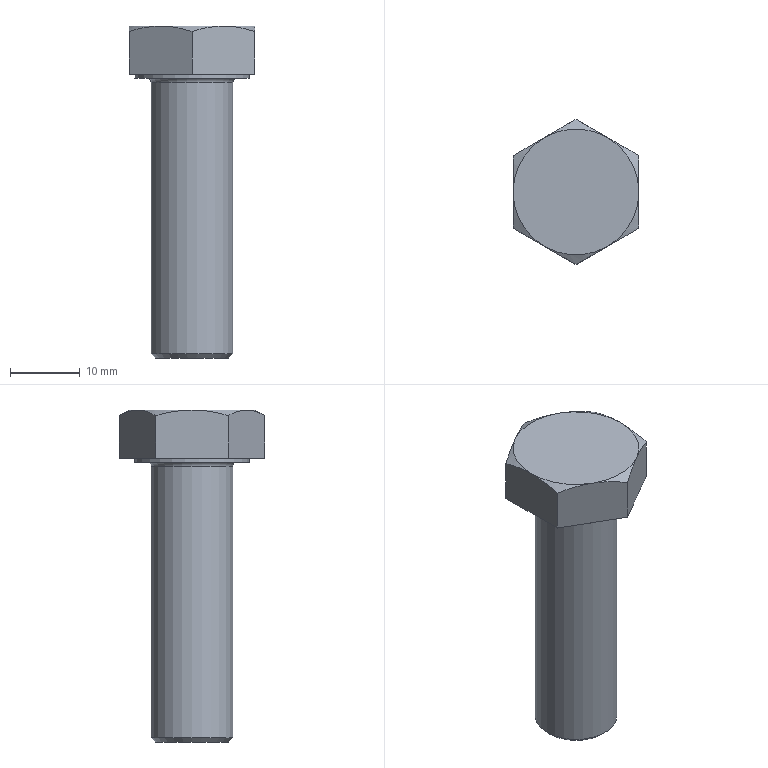Component | NX | GB-T5782-2000_M12X40 | 1 solid | 20 faces | volume 6356 mm3 | plane 10 | cone 7 | cylinder 2 | torus 1 | commonest cylinder face diameters 16.47 x1 11.701 x1